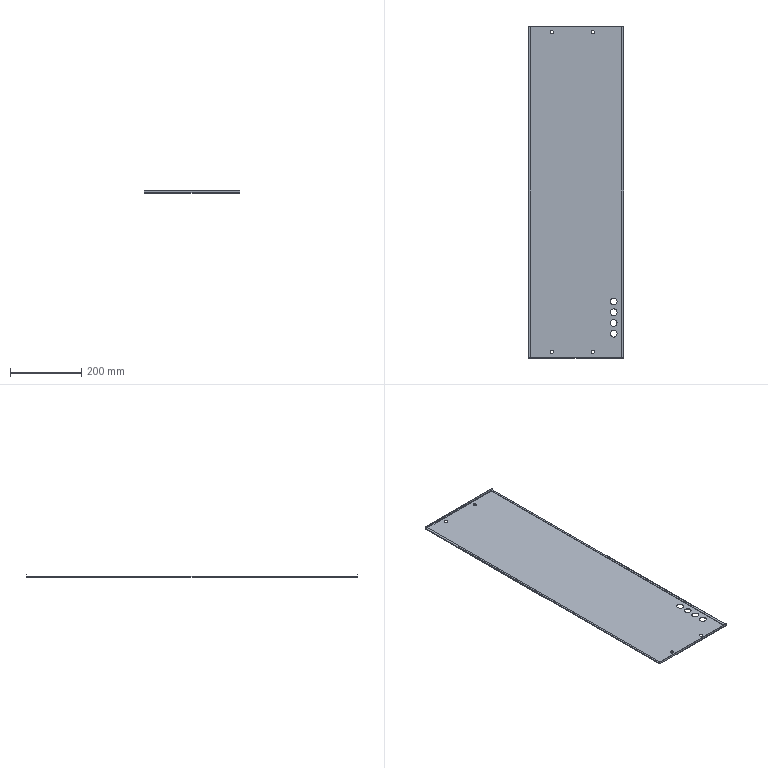Component | SolidWorks | RearCoverPlate100-2 | 1 solid | 58 faces | volume 312435 mm3 | plane 34 | cylinder 24 | commonest cylinder face diameters 10 x8 19 x8 4.8 x2 2.4 x2 2.5 x2 0.1 x2